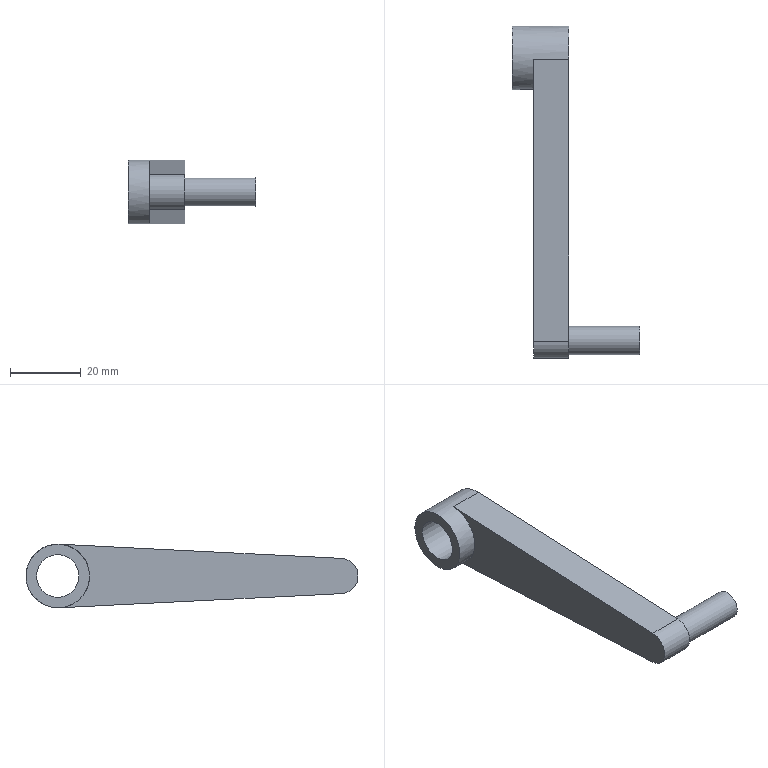Component | NX | HANDLE | 1 solid | 10 faces | box 36 x 94 x 18 mm | volume 13602 mm3 | plane 6 | cylinder 4 | commonest cylinder face diameters 18 x1 12 x1 10 x1 8 x1
STEP:
#1=CARTESIAN_POINT('',(0.,0.,0.));
#2=DIRECTION('',(0.,0.,1.));
#3=DIRECTION('',(1.,0.,0.));
#4=AXIS2_PLACEMENT_3D('',#1,#2,#3);
#5=CARTESIAN_POINT('',(764.009,-150.752,-1316.489));
#6=VERTEX_POINT('',#5);
#7=CARTESIAN_POINT('',(764.009,-159.302,-1307.5));
#8=VERTEX_POINT('',#7);
#9=CARTESIAN_POINT('',(764.009,-150.302,-1307.5));
#10=DIRECTION('',(-1.,0.,0.));
#11=DIRECTION('',(0.,-1.,0.));
#12=AXIS2_PLACEMENT_3D('',#9,#10,#11);
#13=CIRCLE('',#12,9.);
#14=CARTESIAN_POINT('',(764.009,-150.302,-1307.5));
#15=DIRECTION('',(1.,0.,0.));
#16=DIRECTION('',(0.,1.,0.));
#17=AXIS2_PLACEMENT_3D('',#14,#15,#16);
#18=CYLINDRICAL_SURFACE('',#17,9.);
#19=CARTESIAN_POINT('',(15.708,0.));
#20=DIRECTION('',(-1.,0.));
#21=VECTOR('',#20,1.);
#22=LINE('',#19,#21);
#23=(GEOMETRIC_REPRESENTATION_CONTEXT(2)PARAMETRIC_REPRESENTATION_CONTEXT()REPRESENTATION_CONTEXT('',''));
#24=DEFINITIONAL_REPRESENTATION('',(#22),#23);
#25=PCURVE('',#18,#24);
#26=CARTESIAN_POINT('',(764.009,-150.302,-1307.5));
#27=DIRECTION('',(-1.,0.,0.));
#28=DIRECTION('',(0.,-1.,0.));
#29=AXIS2_PLACEMENT_3D('',#26,#27,#28);
#30=PLANE('',#29);
#31=CARTESIAN_POINT('',(0.,0.));
#32=DIRECTION('',(1.,0.));
#33=AXIS2_PLACEMENT_2D('',#31,#32);
#34=CIRCLE('',#33,9.);
#35=(GEOMETRIC_REPRESENTATION_CONTEXT(2)PARAMETRIC_REPRESENTATION_CONTEXT()REPRESENTATION_CONTEXT('',''));
#36=DEFINITIONAL_REPRESENTATION('',(#34),#35);
#37=PCURVE('',#30,#36);
#38=SURFACE_CURVE('',#13,(#25,#37),.PCURVE_S1.);
#39=EDGE_CURVE('',#6,#8,#38,.T.);
#40=ORIENTED_EDGE('',*,*,#39,.F.);
#41=CARTESIAN_POINT('',(770.009,-150.752,-1316.489));
#42=VERTEX_POINT('',#41);
#43=CARTESIAN_POINT('',(764.009,-150.752,-1316.489));
#44=CARTESIAN_POINT('',(770.009,-150.752,-1316.489));
#45=B_SPLINE_CURVE_WITH_KNOTS('',1,(#43,#44),.UNSPECIFIED.,.F.,.F.,(2,2),(0.,6.),.PIECEWISE_BEZIER_KNOTS.);
#46=CARTESIAN_POINT('',(10.946,0.));
#47=DIRECTION('',(0.,1.));
#48=VECTOR('',#47,1.);
#49=LINE('',#46,#48);
#50=(GEOMETRIC_REPRESENTATION_CONTEXT(2)PARAMETRIC_REPRESENTATION_CONTEXT()REPRESENTATION_CONTEXT('',''));
#51=DEFINITIONAL_REPRESENTATION('',(#49),#50);
#52=PCURVE('',#18,#51);
#53=CARTESIAN_POINT('',(4.662,0.));
#54=DIRECTION('',(0.,1.));
#55=VECTOR('',#54,1.);
#56=LINE('',#53,#55);
#57=(GEOMETRIC_REPRESENTATION_CONTEXT(2)PARAMETRIC_REPRESENTATION_CONTEXT()REPRESENTATION_CONTEXT('',''));
#58=DEFINITIONAL_REPRESENTATION('',(#56),#57);
#59=PCURVE('',#18,#58);
#60=SEAM_CURVE('',#45,(#52,#59),.PCURVE_S1.);
#61=EDGE_CURVE('',#6,#42,#60,.T.);
#62=ORIENTED_EDGE('',*,*,#61,.T.);
#63=CARTESIAN_POINT('',(770.009,-150.752,-1298.511));
#64=VERTEX_POINT('',#63);
#65=CARTESIAN_POINT('',(770.009,-150.302,-1307.5));
#66=DIRECTION('',(1.,0.,0.));
#67=DIRECTION('',(0.,-1.,0.));
#68=AXIS2_PLACEMENT_3D('',#65,#66,#67);
#69=CIRCLE('',#68,9.);
#70=CARTESIAN_POINT('',(3.142,6.));
#71=DIRECTION('',(1.,0.));
#72=VECTOR('',#71,1.);
#73=LINE('',#70,#72);
#74=(GEOMETRIC_REPRESENTATION_CONTEXT(2)PARAMETRIC_REPRESENTATION_CONTEXT()REPRESENTATION_CONTEXT('',''));
#75=DEFINITIONAL_REPRESENTATION('',(#73),#74);
#76=PCURVE('',#18,#75);
#77=CARTESIAN_POINT('',(770.009,-150.302,-1307.5));
#78=DIRECTION('',(1.,0.,0.));
#79=DIRECTION('',(0.,1.,0.));
#80=AXIS2_PLACEMENT_3D('',#77,#78,#79);
#81=PLANE('',#80);
#82=CARTESIAN_POINT('',(0.,0.));
#83=DIRECTION('',(-1.,0.));
#84=AXIS2_PLACEMENT_2D('',#82,#83);
#85=CIRCLE('',#84,9.);
#86=(GEOMETRIC_REPRESENTATION_CONTEXT(2)PARAMETRIC_REPRESENTATION_CONTEXT()REPRESENTATION_CONTEXT('',''));
#87=DEFINITIONAL_REPRESENTATION('',(#85),#86);
#88=PCURVE('',#81,#87);
#89=SURFACE_CURVE('',#69,(#76,#88),.PCURVE_S1.);
#90=EDGE_CURVE('',#64,#42,#89,.T.);
#91=ORIENTED_EDGE('',*,*,#90,.F.);
#92=CARTESIAN_POINT('',(780.009,-150.752,-1298.511));
#93=VERTEX_POINT('',#92);
#94=CARTESIAN_POINT('',(770.009,-150.752,-1298.511));
#95=DIRECTION('',(1.,0.,0.));
#96=VECTOR('',#95,1.);
#97=LINE('',#94,#96);
#98=CARTESIAN_POINT('',(7.904,6.));
#99=DIRECTION('',(0.,1.));
#100=VECTOR('',#99,1.);
#101=LINE('',#98,#100);
#102=(GEOMETRIC_REPRESENTATION_CONTEXT(2)PARAMETRIC_REPRESENTATION_CONTEXT()REPRESENTATION_CONTEXT('',''));
#103=DEFINITIONAL_REPRESENTATION('',(#101),#102);
#104=PCURVE('',#18,#103);
#105=CARTESIAN_POINT('',(770.009,-230.552,-1302.506));
#106=DIRECTION('',(0.,0.05,-0.9987));
#107=DIRECTION('',(0.,-0.9987,-0.05));
#108=AXIS2_PLACEMENT_3D('',#105,#106,#107);
#109=PLANE('',#108);
#110=CARTESIAN_POINT('',(-79.9,0.));
#111=DIRECTION('',(0.,-1.));
#112=VECTOR('',#111,1.);
#113=LINE('',#110,#112);
#114=(GEOMETRIC_REPRESENTATION_CONTEXT(2)PARAMETRIC_REPRESENTATION_CONTEXT()REPRESENTATION_CONTEXT('',''));
#115=DEFINITIONAL_REPRESENTATION('',(#113),#114);
#116=PCURVE('',#109,#115);
#117=SURFACE_CURVE('',#97,(#104,#116),.PCURVE_S1.);
#118=EDGE_CURVE('',#64,#93,#117,.T.);
#119=ORIENTED_EDGE('',*,*,#118,.T.);
#120=CARTESIAN_POINT('',(780.009,-150.752,-1316.489));
#121=VERTEX_POINT('',#120);
#122=CARTESIAN_POINT('',(780.009,-150.302,-1307.5));
#123=DIRECTION('',(-1.,0.,0.));
#124=DIRECTION('',(0.,-1.,0.));
#125=AXIS2_PLACEMENT_3D('',#122,#123,#124);
#126=CIRCLE('',#125,9.);
#127=CARTESIAN_POINT('',(9.425,16.));
#128=DIRECTION('',(-1.,0.));
#129=VECTOR('',#128,1.);
#130=LINE('',#127,#129);
#131=(GEOMETRIC_REPRESENTATION_CONTEXT(2)PARAMETRIC_REPRESENTATION_CONTEXT()REPRESENTATION_CONTEXT('',''));
#132=DEFINITIONAL_REPRESENTATION('',(#130),#131);
#133=PCURVE('',#18,#132);
#134=CARTESIAN_POINT('',(780.009,-150.302,-1307.5));
#135=DIRECTION('',(-1.,0.,0.));
#136=DIRECTION('',(0.,-1.,0.));
#137=AXIS2_PLACEMENT_3D('',#134,#135,#136);
#138=PLANE('',#137);
#139=CARTESIAN_POINT('',(0.,0.));
#140=DIRECTION('',(1.,0.));
#141=AXIS2_PLACEMENT_2D('',#139,#140);
#142=CIRCLE('',#141,9.);
#143=(GEOMETRIC_REPRESENTATION_CONTEXT(2)PARAMETRIC_REPRESENTATION_CONTEXT()REPRESENTATION_CONTEXT('',''));
#144=DEFINITIONAL_REPRESENTATION('',(#142),#143);
#145=PCURVE('',#138,#144);
#146=SURFACE_CURVE('',#126,(#133,#145),.PCURVE_S1.);
#147=EDGE_CURVE('',#93,#121,#146,.T.);
#148=ORIENTED_EDGE('',*,*,#147,.T.);
#149=CARTESIAN_POINT('',(770.009,-150.752,-1316.489));
#150=DIRECTION('',(1.,0.,0.));
#151=VECTOR('',#150,1.);
#152=LINE('',#149,#151);
#153=CARTESIAN_POINT('',(4.662,6.));
#154=DIRECTION('',(0.,1.));
#155=VECTOR('',#154,1.);
#156=LINE('',#153,#155);
#157=(GEOMETRIC_REPRESENTATION_CONTEXT(2)PARAMETRIC_REPRESENTATION_CONTEXT()REPRESENTATION_CONTEXT('',''));
#158=DEFINITIONAL_REPRESENTATION('',(#156),#157);
#159=PCURVE('',#18,#158);
#160=CARTESIAN_POINT('',(770.009,-150.752,-1316.489));
#161=DIRECTION('',(0.,0.05,0.9987));
#162=DIRECTION('',(0.,0.9987,-0.05));
#163=AXIS2_PLACEMENT_3D('',#160,#161,#162);
#164=PLANE('',#163);
#165=CARTESIAN_POINT('',(-0.,0.));
#166=DIRECTION('',(0.,-1.));
#167=VECTOR('',#166,1.);
#168=LINE('',#165,#167);
#169=(GEOMETRIC_REPRESENTATION_CONTEXT(2)PARAMETRIC_REPRESENTATION_CONTEXT()REPRESENTATION_CONTEXT('',''));
#170=DEFINITIONAL_REPRESENTATION('',(#168),#169);
#171=PCURVE('',#164,#170);
#172=SURFACE_CURVE('',#152,(#159,#171),.PCURVE_S1.);
#173=EDGE_CURVE('',#42,#121,#172,.T.);
#174=ORIENTED_EDGE('',*,*,#173,.F.);
#175=ORIENTED_EDGE('',*,*,#61,.F.);
#176=CARTESIAN_POINT('',(764.009,-150.302,-1307.5));
#177=DIRECTION('',(-1.,0.,0.));
#178=DIRECTION('',(0.,-1.,0.));
#179=AXIS2_PLACEMENT_3D('',#176,#177,#178);
#180=CIRCLE('',#179,9.);
#181=CARTESIAN_POINT('',(9.425,0.));
#182=DIRECTION('',(-1.,0.));
#183=VECTOR('',#182,1.);
#184=LINE('',#181,#183);
#185=(GEOMETRIC_REPRESENTATION_CONTEXT(2)PARAMETRIC_REPRESENTATION_CONTEXT()REPRESENTATION_CONTEXT('',''));
#186=DEFINITIONAL_REPRESENTATION('',(#184),#185);
#187=PCURVE('',#18,#186);
#188=CARTESIAN_POINT('',(0.,0.));
#189=DIRECTION('',(1.,0.));
#190=AXIS2_PLACEMENT_2D('',#188,#189);
#191=CIRCLE('',#190,9.);
#192=(GEOMETRIC_REPRESENTATION_CONTEXT(2)PARAMETRIC_REPRESENTATION_CONTEXT()REPRESENTATION_CONTEXT('',''));
#193=DEFINITIONAL_REPRESENTATION('',(#191),#192);
#194=PCURVE('',#30,#193);
#195=SURFACE_CURVE('',#180,(#187,#194),.PCURVE_S1.);
#196=EDGE_CURVE('',#8,#6,#195,.T.);
#197=ORIENTED_EDGE('',*,*,#196,.F.);
#198=EDGE_LOOP('',(#40,#62,#91,#119,#148,#174,#175,#197));
#199=FACE_BOUND('',#198,.T.);
#200=ADVANCED_FACE('',(#199),#18,.T.);
#201=CARTESIAN_POINT('',(764.009,-156.302,-1307.5));
#202=VERTEX_POINT('',#201);
#203=CARTESIAN_POINT('',(764.009,-150.302,-1307.5));
#204=DIRECTION('',(-1.,0.,0.));
#205=DIRECTION('',(0.,-1.,0.));
#206=AXIS2_PLACEMENT_3D('',#203,#204,#205);
#207=CIRCLE('',#206,6.);
#208=CARTESIAN_POINT('',(764.009,-150.302,-1307.5));
#209=DIRECTION('',(1.,0.,0.));
#210=DIRECTION('',(0.,1.,0.));
#211=AXIS2_PLACEMENT_3D('',#208,#209,#210);
#212=CYLINDRICAL_SURFACE('',#211,6.);
#213=CARTESIAN_POINT('',(9.425,0.));
#214=DIRECTION('',(-1.,0.));
#215=VECTOR('',#214,1.);
#216=LINE('',#213,#215);
#217=(GEOMETRIC_REPRESENTATION_CONTEXT(2)PARAMETRIC_REPRESENTATION_CONTEXT()REPRESENTATION_CONTEXT('',''));
#218=DEFINITIONAL_REPRESENTATION('',(#216),#217);
#219=PCURVE('',#212,#218);
#220=CARTESIAN_POINT('',(0.,0.));
#221=DIRECTION('',(1.,0.));
#222=AXIS2_PLACEMENT_2D('',#220,#221);
#223=CIRCLE('',#222,6.);
#224=(GEOMETRIC_REPRESENTATION_CONTEXT(2)PARAMETRIC_REPRESENTATION_CONTEXT()REPRESENTATION_CONTEXT('',''));
#225=DEFINITIONAL_REPRESENTATION('',(#223),#224);
#226=PCURVE('',#30,#225);
#227=SURFACE_CURVE('',#207,(#219,#226),.PCURVE_S1.);
#228=EDGE_CURVE('',#202,#202,#227,.T.);
#229=ORIENTED_EDGE('',*,*,#228,.F.);
#230=CARTESIAN_POINT('',(780.009,-156.302,-1307.5));
#231=VERTEX_POINT('',#230);
#232=CARTESIAN_POINT('',(764.009,-156.302,-1307.5));
#233=CARTESIAN_POINT('',(780.009,-156.302,-1307.5));
#234=B_SPLINE_CURVE_WITH_KNOTS('',1,(#232,#233),.UNSPECIFIED.,.F.,.F.,(2,2),(0.,16.),.PIECEWISE_BEZIER_KNOTS.);
#235=CARTESIAN_POINT('',(9.425,0.));
#236=DIRECTION('',(0.,1.));
#237=VECTOR('',#236,1.);
#238=LINE('',#235,#237);
#239=(GEOMETRIC_REPRESENTATION_CONTEXT(2)PARAMETRIC_REPRESENTATION_CONTEXT()REPRESENTATION_CONTEXT('',''));
#240=DEFINITIONAL_REPRESENTATION('',(#238),#239);
#241=PCURVE('',#212,#240);
#242=CARTESIAN_POINT('',(3.142,0.));
#243=DIRECTION('',(0.,1.));
#244=VECTOR('',#243,1.);
#245=LINE('',#242,#244);
#246=(GEOMETRIC_REPRESENTATION_CONTEXT(2)PARAMETRIC_REPRESENTATION_CONTEXT()REPRESENTATION_CONTEXT('',''));
#247=DEFINITIONAL_REPRESENTATION('',(#245),#246);
#248=PCURVE('',#212,#247);
#249=SEAM_CURVE('',#234,(#241,#248),.PCURVE_S1.);
#250=EDGE_CURVE('',#202,#231,#249,.T.);
#251=ORIENTED_EDGE('',*,*,#250,.T.);
#252=CARTESIAN_POINT('',(780.009,-150.302,-1307.5));
#253=DIRECTION('',(-1.,0.,0.));
#254=DIRECTION('',(0.,-1.,0.));
#255=AXIS2_PLACEMENT_3D('',#252,#253,#254);
#256=CIRCLE('',#255,6.);
#257=CARTESIAN_POINT('',(9.425,16.));
#258=DIRECTION('',(-1.,0.));
#259=VECTOR('',#258,1.);
#260=LINE('',#257,#259);
#261=(GEOMETRIC_REPRESENTATION_CONTEXT(2)PARAMETRIC_REPRESENTATION_CONTEXT()REPRESENTATION_CONTEXT('',''));
#262=DEFINITIONAL_REPRESENTATION('',(#260),#261);
#263=PCURVE('',#212,#262);
#264=CARTESIAN_POINT('',(0.,0.));
#265=DIRECTION('',(1.,0.));
#266=AXIS2_PLACEMENT_2D('',#264,#265);
#267=CIRCLE('',#266,6.);
#268=(GEOMETRIC_REPRESENTATION_CONTEXT(2)PARAMETRIC_REPRESENTATION_CONTEXT()REPRESENTATION_CONTEXT('',''));
#269=DEFINITIONAL_REPRESENTATION('',(#267),#268);
#270=PCURVE('',#138,#269);
#271=SURFACE_CURVE('',#256,(#263,#270),.PCURVE_S1.);
#272=EDGE_CURVE('',#231,#231,#271,.T.);
#273=ORIENTED_EDGE('',*,*,#272,.T.);
#274=ORIENTED_EDGE('',*,*,#250,.F.);
#275=EDGE_LOOP('',(#229,#251,#273,#274));
#276=FACE_BOUND('',#275,.F.);
#277=ADVANCED_FACE('',(#276),#212,.F.);
#278=ORIENTED_EDGE('',*,*,#196,.T.);
#279=ORIENTED_EDGE('',*,*,#39,.T.);
#280=EDGE_LOOP('',(#278,#279));
#281=FACE_BOUND('',#280,.T.);
#282=ORIENTED_EDGE('',*,*,#228,.F.);
#283=EDGE_LOOP('',(#282));
#284=FACE_BOUND('',#283,.T.);
#285=ADVANCED_FACE('',(#281,#284),#30,.T.);
#286=CARTESIAN_POINT('',(780.009,-234.302,-1307.5));
#287=VERTEX_POINT('',#286);
#288=CARTESIAN_POINT('',(780.009,-230.302,-1307.5));
#289=DIRECTION('',(1.,0.,0.));
#290=DIRECTION('',(0.,-1.,0.));
#291=AXIS2_PLACEMENT_3D('',#288,#289,#290);
#292=CIRCLE('',#291,4.);
#293=CARTESIAN_POINT('',(84.,0.));
#294=CARTESIAN_POINT('',(84.,-6.928));
#295=CARTESIAN_POINT('',(78.,-3.464));
#296=CARTESIAN_POINT('',(72.,-0.));
#297=CARTESIAN_POINT('',(78.,3.464));
#298=CARTESIAN_POINT('',(84.,6.928));
#299=CARTESIAN_POINT('',(84.,0.));
#300=(BOUNDED_CURVE()B_SPLINE_CURVE(2,(#293,#294,#295,#296,#297,#298,#299),.UNSPECIFIED.,.T.,.F.)B_SPLINE_CURVE_WITH_KNOTS((1,2,2,2,2,1),(-2.094,0.,2.094,4.189,6.283,8.378),.UNSPECIFIED.)CURVE()GEOMETRIC_REPRESENTATION_ITEM()RATIONAL_B_SPLINE_CURVE((1.,0.5,1.,0.5,1.,0.5,1.))REPRESENTATION_ITEM(''));
#301=(GEOMETRIC_REPRESENTATION_CONTEXT(2)PARAMETRIC_REPRESENTATION_CONTEXT()REPRESENTATION_CONTEXT('',''));
#302=DEFINITIONAL_REPRESENTATION('',(#300),#301);
#303=PCURVE('',#138,#302);
#304=CARTESIAN_POINT('',(800.009,-230.302,-1307.5));
#305=DIRECTION('',(-1.,0.,0.));
#306=DIRECTION('',(0.,-1.,0.));
#307=AXIS2_PLACEMENT_3D('',#304,#305,#306);
#308=CYLINDRICAL_SURFACE('',#307,4.);
#309=CARTESIAN_POINT('',(6.283,20.));
#310=DIRECTION('',(-1.,0.));
#311=VECTOR('',#310,1.);
#312=LINE('',#309,#311);
#313=(GEOMETRIC_REPRESENTATION_CONTEXT(2)PARAMETRIC_REPRESENTATION_CONTEXT()REPRESENTATION_CONTEXT('',''));
#314=DEFINITIONAL_REPRESENTATION('',(#312),#313);
#315=PCURVE('',#308,#314);
#316=SURFACE_CURVE('',#292,(#303,#315),.PCURVE_S1.);
#317=EDGE_CURVE('',#287,#287,#316,.T.);
#318=ORIENTED_EDGE('',*,*,#317,.F.);
#319=EDGE_LOOP('',(#318));
#320=FACE_BOUND('',#319,.T.);
#321=ORIENTED_EDGE('',*,*,#147,.F.);
#322=CARTESIAN_POINT('',(780.009,-230.552,-1302.506));
#323=VERTEX_POINT('',#322);
#324=CARTESIAN_POINT('',(780.009,-230.552,-1302.506));
#325=DIRECTION('',(0.,0.9987,0.05));
#326=VECTOR('',#325,1.);
#327=LINE('',#324,#326);
#328=CARTESIAN_POINT('',(80.25,4.994));
#329=DIRECTION('',(-0.9987,0.05));
#330=VECTOR('',#329,1.);
#331=LINE('',#328,#330);
#332=(GEOMETRIC_REPRESENTATION_CONTEXT(2)PARAMETRIC_REPRESENTATION_CONTEXT()REPRESENTATION_CONTEXT('',''));
#333=DEFINITIONAL_REPRESENTATION('',(#331),#332);
#334=PCURVE('',#138,#333);
#335=CARTESIAN_POINT('',(0.,-10.));
#336=DIRECTION('',(-1.,0.));
#337=VECTOR('',#336,1.);
#338=LINE('',#335,#337);
#339=(GEOMETRIC_REPRESENTATION_CONTEXT(2)PARAMETRIC_REPRESENTATION_CONTEXT()REPRESENTATION_CONTEXT('',''));
#340=DEFINITIONAL_REPRESENTATION('',(#338),#339);
#341=PCURVE('',#109,#340);
#342=SURFACE_CURVE('',#327,(#334,#341),.PCURVE_S1.);
#343=EDGE_CURVE('',#323,#93,#342,.T.);
#344=ORIENTED_EDGE('',*,*,#343,.F.);
#345=CARTESIAN_POINT('',(780.009,-230.552,-1312.494));
#346=VERTEX_POINT('',#345);
#347=CARTESIAN_POINT('',(780.009,-230.302,-1307.5));
#348=DIRECTION('',(-1.,0.,0.));
#349=DIRECTION('',(0.,-1.,0.));
#350=AXIS2_PLACEMENT_3D('',#347,#348,#349);
#351=CIRCLE('',#350,5.);
#352=CARTESIAN_POINT('',(80.,0.));
#353=DIRECTION('',(1.,0.));
#354=AXIS2_PLACEMENT_2D('',#352,#353);
#355=CIRCLE('',#354,5.);
#356=(GEOMETRIC_REPRESENTATION_CONTEXT(2)PARAMETRIC_REPRESENTATION_CONTEXT()REPRESENTATION_CONTEXT('',''));
#357=DEFINITIONAL_REPRESENTATION('',(#355),#356);
#358=PCURVE('',#138,#357);
#359=CARTESIAN_POINT('',(770.009,-230.302,-1307.5));
#360=DIRECTION('',(1.,0.,0.));
#361=DIRECTION('',(0.,1.,0.));
#362=AXIS2_PLACEMENT_3D('',#359,#360,#361);
#363=CYLINDRICAL_SURFACE('',#362,5.);
#364=CARTESIAN_POINT('',(9.425,10.));
#365=DIRECTION('',(-1.,0.));
#366=VECTOR('',#365,1.);
#367=LINE('',#364,#366);
#368=(GEOMETRIC_REPRESENTATION_CONTEXT(2)PARAMETRIC_REPRESENTATION_CONTEXT()REPRESENTATION_CONTEXT('',''));
#369=DEFINITIONAL_REPRESENTATION('',(#367),#368);
#370=PCURVE('',#363,#369);
#371=SURFACE_CURVE('',#351,(#358,#370),.PCURVE_S1.);
#372=EDGE_CURVE('',#346,#323,#371,.T.);
#373=ORIENTED_EDGE('',*,*,#372,.F.);
#374=CARTESIAN_POINT('',(780.009,-150.752,-1316.489));
#375=DIRECTION('',(0.,-0.9987,0.05));
#376=VECTOR('',#375,1.);
#377=LINE('',#374,#376);
#378=CARTESIAN_POINT('',(0.45,-8.989));
#379=DIRECTION('',(0.9987,0.05));
#380=VECTOR('',#379,1.);
#381=LINE('',#378,#380);
#382=(GEOMETRIC_REPRESENTATION_CONTEXT(2)PARAMETRIC_REPRESENTATION_CONTEXT()REPRESENTATION_CONTEXT('',''));
#383=DEFINITIONAL_REPRESENTATION('',(#381),#382);
#384=PCURVE('',#138,#383);
#385=CARTESIAN_POINT('',(0.,-10.));
#386=DIRECTION('',(-1.,0.));
#387=VECTOR('',#386,1.);
#388=LINE('',#385,#387);
#389=(GEOMETRIC_REPRESENTATION_CONTEXT(2)PARAMETRIC_REPRESENTATION_CONTEXT()REPRESENTATION_CONTEXT('',''));
#390=DEFINITIONAL_REPRESENTATION('',(#388),#389);
#391=PCURVE('',#164,#390);
#392=SURFACE_CURVE('',#377,(#384,#391),.PCURVE_S1.);
#393=EDGE_CURVE('',#121,#346,#392,.T.);
#394=ORIENTED_EDGE('',*,*,#393,.F.);
#395=EDGE_LOOP('',(#321,#344,#373,#394));
#396=FACE_BOUND('',#395,.T.);
#397=ORIENTED_EDGE('',*,*,#272,.T.);
#398=EDGE_LOOP('',(#397));
#399=FACE_BOUND('',#398,.T.);
#400=ADVANCED_FACE('',(#320,#396,#399),#138,.F.);
#401=ORIENTED_EDGE('',*,*,#393,.T.);
#402=CARTESIAN_POINT('',(770.009,-230.552,-1312.494));
#403=VERTEX_POINT('',#402);
#404=CARTESIAN_POINT('',(770.009,-230.552,-1312.494));
#405=DIRECTION('',(1.,0.,0.));
#406=VECTOR('',#405,1.);
#407=LINE('',#404,#406);
#408=CARTESIAN_POINT('',(-79.9,0.));
#409=DIRECTION('',(0.,-1.));
#410=VECTOR('',#409,1.);
#411=LINE('',#408,#410);
#412=(GEOMETRIC_REPRESENTATION_CONTEXT(2)PARAMETRIC_REPRESENTATION_CONTEXT()REPRESENTATION_CONTEXT('',''));
#413=DEFINITIONAL_REPRESENTATION('',(#411),#412);
#414=PCURVE('',#164,#413);
#415=CARTESIAN_POINT('',(4.662,0.));
#416=DIRECTION('',(0.,1.));
#417=VECTOR('',#416,1.);
#418=LINE('',#415,#417);
#419=(GEOMETRIC_REPRESENTATION_CONTEXT(2)PARAMETRIC_REPRESENTATION_CONTEXT()REPRESENTATION_CONTEXT('',''));
#420=DEFINITIONAL_REPRESENTATION('',(#418),#419);
#421=PCURVE('',#363,#420);
#422=SURFACE_CURVE('',#407,(#414,#421),.PCURVE_S1.);
#423=EDGE_CURVE('',#403,#346,#422,.T.);
#424=ORIENTED_EDGE('',*,*,#423,.F.);
#425=CARTESIAN_POINT('',(770.009,-150.752,-1316.489));
#426=DIRECTION('',(0.,-0.9987,0.05));
#427=VECTOR('',#426,1.);
#428=LINE('',#425,#427);
#429=CARTESIAN_POINT('',(0.,0.));
#430=DIRECTION('',(-1.,0.));
#431=VECTOR('',#430,1.);
#432=LINE('',#429,#431);
#433=(GEOMETRIC_REPRESENTATION_CONTEXT(2)PARAMETRIC_REPRESENTATION_CONTEXT()REPRESENTATION_CONTEXT('',''));
#434=DEFINITIONAL_REPRESENTATION('',(#432),#433);
#435=PCURVE('',#164,#434);
#436=CARTESIAN_POINT('',(-0.45,-8.989));
#437=DIRECTION('',(-0.9987,0.05));
#438=VECTOR('',#437,1.);
#439=LINE('',#436,#438);
#440=(GEOMETRIC_REPRESENTATION_CONTEXT(2)PARAMETRIC_REPRESENTATION_CONTEXT()REPRESENTATION_CONTEXT('',''));
#441=DEFINITIONAL_REPRESENTATION('',(#439),#440);
#442=PCURVE('',#81,#441);
#443=SURFACE_CURVE('',#428,(#435,#442),.PCURVE_S1.);
#444=EDGE_CURVE('',#42,#403,#443,.T.);
#445=ORIENTED_EDGE('',*,*,#444,.F.);
#446=ORIENTED_EDGE('',*,*,#173,.T.);
#447=EDGE_LOOP('',(#401,#424,#445,#446));
#448=FACE_BOUND('',#447,.T.);
#449=ADVANCED_FACE('',(#448),#164,.F.);
#450=ORIENTED_EDGE('',*,*,#372,.T.);
#451=CARTESIAN_POINT('',(770.009,-230.552,-1302.506));
#452=VERTEX_POINT('',#451);
#453=CARTESIAN_POINT('',(770.009,-230.552,-1302.506));
#454=DIRECTION('',(1.,0.,0.));
#455=VECTOR('',#454,1.);
#456=LINE('',#453,#455);
#457=CARTESIAN_POINT('',(1.621,0.));
#458=DIRECTION('',(0.,1.));
#459=VECTOR('',#458,1.);
#460=LINE('',#457,#459);
#461=(GEOMETRIC_REPRESENTATION_CONTEXT(2)PARAMETRIC_REPRESENTATION_CONTEXT()REPRESENTATION_CONTEXT('',''));
#462=DEFINITIONAL_REPRESENTATION('',(#460),#461);
#463=PCURVE('',#363,#462);
#464=CARTESIAN_POINT('',(0.,0.));
#465=DIRECTION('',(0.,-1.));
#466=VECTOR('',#465,1.);
#467=LINE('',#464,#466);
#468=(GEOMETRIC_REPRESENTATION_CONTEXT(2)PARAMETRIC_REPRESENTATION_CONTEXT()REPRESENTATION_CONTEXT('',''));
#469=DEFINITIONAL_REPRESENTATION('',(#467),#468);
#470=PCURVE('',#109,#469);
#471=SURFACE_CURVE('',#456,(#463,#470),.PCURVE_S1.);
#472=EDGE_CURVE('',#452,#323,#471,.T.);
#473=ORIENTED_EDGE('',*,*,#472,.F.);
#474=CARTESIAN_POINT('',(770.009,-230.302,-1307.5));
#475=DIRECTION('',(-1.,0.,0.));
#476=DIRECTION('',(0.,-1.,0.));
#477=AXIS2_PLACEMENT_3D('',#474,#475,#476);
#478=CIRCLE('',#477,5.);
#479=CARTESIAN_POINT('',(9.425,0.));
#480=DIRECTION('',(-1.,0.));
#481=VECTOR('',#480,1.);
#482=LINE('',#479,#481);
#483=(GEOMETRIC_REPRESENTATION_CONTEXT(2)PARAMETRIC_REPRESENTATION_CONTEXT()REPRESENTATION_CONTEXT('',''));
#484=DEFINITIONAL_REPRESENTATION('',(#482),#483);
#485=PCURVE('',#363,#484);
#486=CARTESIAN_POINT('',(-85.,0.));
#487=CARTESIAN_POINT('',(-85.,8.66));
#488=CARTESIAN_POINT('',(-77.5,4.33));
#489=CARTESIAN_POINT('',(-70.,0.));
#490=CARTESIAN_POINT('',(-77.5,-4.33));
#491=CARTESIAN_POINT('',(-85.,-8.66));
#492=CARTESIAN_POINT('',(-85.,0.));
#493=(BOUNDED_CURVE()B_SPLINE_CURVE(2,(#486,#487,#488,#489,#490,#491,#492),.UNSPECIFIED.,.T.,.F.)B_SPLINE_CURVE_WITH_KNOTS((1,2,2,2,2,1),(-2.094,0.,2.094,4.189,6.283,8.378),.UNSPECIFIED.)CURVE()GEOMETRIC_REPRESENTATION_ITEM()RATIONAL_B_SPLINE_CURVE((1.,0.5,1.,0.5,1.,0.5,1.))REPRESENTATION_ITEM(''));
#494=(GEOMETRIC_REPRESENTATION_CONTEXT(2)PARAMETRIC_REPRESENTATION_CONTEXT()REPRESENTATION_CONTEXT('',''));
#495=DEFINITIONAL_REPRESENTATION('',(#493),#494);
#496=PCURVE('',#81,#495);
#497=SURFACE_CURVE('',#478,(#485,#496),.PCURVE_S1.);
#498=EDGE_CURVE('',#403,#452,#497,.T.);
#499=ORIENTED_EDGE('',*,*,#498,.F.);
#500=ORIENTED_EDGE('',*,*,#423,.T.);
#501=EDGE_LOOP('',(#450,#473,#499,#500));
#502=FACE_BOUND('',#501,.T.);
#503=ADVANCED_FACE('',(#502),#363,.T.);
#504=ORIENTED_EDGE('',*,*,#343,.T.);
#505=ORIENTED_EDGE('',*,*,#118,.F.);
#506=CARTESIAN_POINT('',(770.009,-230.552,-1302.506));
#507=DIRECTION('',(0.,0.9987,0.05));
#508=VECTOR('',#507,1.);
#509=LINE('',#506,#508);
#510=CARTESIAN_POINT('',(0.,0.));
#511=DIRECTION('',(-1.,0.));
#512=VECTOR('',#511,1.);
#513=LINE('',#510,#512);
#514=(GEOMETRIC_REPRESENTATION_CONTEXT(2)PARAMETRIC_REPRESENTATION_CONTEXT()REPRESENTATION_CONTEXT('',''));
#515=DEFINITIONAL_REPRESENTATION('',(#513),#514);
#516=PCURVE('',#109,#515);
#517=CARTESIAN_POINT('',(-80.25,4.994));
#518=DIRECTION('',(0.9987,0.05));
#519=VECTOR('',#518,1.);
#520=LINE('',#517,#519);
#521=(GEOMETRIC_REPRESENTATION_CONTEXT(2)PARAMETRIC_REPRESENTATION_CONTEXT()REPRESENTATION_CONTEXT('',''));
#522=DEFINITIONAL_REPRESENTATION('',(#520),#521);
#523=PCURVE('',#81,#522);
#524=SURFACE_CURVE('',#509,(#516,#523),.PCURVE_S1.);
#525=EDGE_CURVE('',#452,#64,#524,.T.);
#526=ORIENTED_EDGE('',*,*,#525,.F.);
#527=ORIENTED_EDGE('',*,*,#472,.T.);
#528=EDGE_LOOP('',(#504,#505,#526,#527));
#529=FACE_BOUND('',#528,.T.);
#530=ADVANCED_FACE('',(#529),#109,.F.);
#531=ORIENTED_EDGE('',*,*,#90,.T.);
#532=ORIENTED_EDGE('',*,*,#444,.T.);
#533=ORIENTED_EDGE('',*,*,#498,.T.);
#534=ORIENTED_EDGE('',*,*,#525,.T.);
#535=EDGE_LOOP('',(#531,#532,#533,#534));
#536=FACE_BOUND('',#535,.T.);
#537=ADVANCED_FACE('',(#536),#81,.F.);
#538=CARTESIAN_POINT('',(800.009,-234.302,-1307.5));
#539=VERTEX_POINT('',#538);
#540=CARTESIAN_POINT('',(800.009,-230.302,-1307.5));
#541=DIRECTION('',(1.,0.,0.));
#542=DIRECTION('',(0.,-1.,0.));
#543=AXIS2_PLACEMENT_3D('',#540,#541,#542);
#544=CIRCLE('',#543,4.);
#545=CARTESIAN_POINT('',(6.283,0.));
#546=DIRECTION('',(-1.,0.));
#547=VECTOR('',#546,1.);
#548=LINE('',#545,#547);
#549=(GEOMETRIC_REPRESENTATION_CONTEXT(2)PARAMETRIC_REPRESENTATION_CONTEXT()REPRESENTATION_CONTEXT('',''));
#550=DEFINITIONAL_REPRESENTATION('',(#548),#549);
#551=PCURVE('',#308,#550);
#552=CARTESIAN_POINT('',(800.009,-230.302,-1307.5));
#553=DIRECTION('',(1.,0.,0.));
#554=DIRECTION('',(0.,1.,0.));
#555=AXIS2_PLACEMENT_3D('',#552,#553,#554);
#556=PLANE('',#555);
#557=CARTESIAN_POINT('',(0.,0.));
#558=DIRECTION('',(-1.,0.));
#559=AXIS2_PLACEMENT_2D('',#557,#558);
#560=CIRCLE('',#559,4.);
#561=(GEOMETRIC_REPRESENTATION_CONTEXT(2)PARAMETRIC_REPRESENTATION_CONTEXT()REPRESENTATION_CONTEXT('',''));
#562=DEFINITIONAL_REPRESENTATION('',(#560),#561);
#563=PCURVE('',#556,#562);
#564=SURFACE_CURVE('',#544,(#551,#563),.PCURVE_S1.);
#565=EDGE_CURVE('',#539,#539,#564,.T.);
#566=ORIENTED_EDGE('',*,*,#565,.F.);
#567=CARTESIAN_POINT('',(800.009,-234.302,-1307.5));
#568=CARTESIAN_POINT('',(780.009,-234.302,-1307.5));
#569=B_SPLINE_CURVE_WITH_KNOTS('',1,(#567,#568),.UNSPECIFIED.,.F.,.F.,(2,2),(0.,20.),.PIECEWISE_BEZIER_KNOTS.);
#570=CARTESIAN_POINT('',(6.283,0.));
#571=DIRECTION('',(0.,1.));
#572=VECTOR('',#571,1.);
#573=LINE('',#570,#572);
#574=(GEOMETRIC_REPRESENTATION_CONTEXT(2)PARAMETRIC_REPRESENTATION_CONTEXT()REPRESENTATION_CONTEXT('',''));
#575=DEFINITIONAL_REPRESENTATION('',(#573),#574);
#576=PCURVE('',#308,#575);
#577=CARTESIAN_POINT('',(0.,0.));
#578=DIRECTION('',(0.,1.));
#579=VECTOR('',#578,1.);
#580=LINE('',#577,#579);
#581=(GEOMETRIC_REPRESENTATION_CONTEXT(2)PARAMETRIC_REPRESENTATION_CONTEXT()REPRESENTATION_CONTEXT('',''));
#582=DEFINITIONAL_REPRESENTATION('',(#580),#581);
#583=PCURVE('',#308,#582);
#584=SEAM_CURVE('',#569,(#576,#583),.PCURVE_S1.);
#585=EDGE_CURVE('',#539,#287,#584,.T.);
#586=ORIENTED_EDGE('',*,*,#585,.T.);
#587=ORIENTED_EDGE('',*,*,#317,.T.);
#588=ORIENTED_EDGE('',*,*,#585,.F.);
#589=EDGE_LOOP('',(#566,#586,#587,#588));
#590=FACE_BOUND('',#589,.T.);
#591=ADVANCED_FACE('',(#590),#308,.T.);
#592=ORIENTED_EDGE('',*,*,#565,.T.);
#593=EDGE_LOOP('',(#592));
#594=FACE_BOUND('',#593,.T.);
#595=ADVANCED_FACE('',(#594),#556,.T.);
#596=CLOSED_SHELL('',(#200,#277,#285,#400,#449,#503,#530,#537,#591,#595));
#597=MANIFOLD_SOLID_BREP('',#596);
#598=(LENGTH_UNIT()NAMED_UNIT(*)SI_UNIT(.MILLI.,.METRE.));
#599=UNCERTAINTY_MEASURE_WITH_UNIT(LENGTH_MEASURE(0.000002),#598,'','');
#600=(NAMED_UNIT(*)PLANE_ANGLE_UNIT()SI_UNIT($,.RADIAN.));
#601=(NAMED_UNIT(*)SI_UNIT($,.STERADIAN.)SOLID_ANGLE_UNIT());
#602=(GEOMETRIC_REPRESENTATION_CONTEXT(3)GLOBAL_UNCERTAINTY_ASSIGNED_CONTEXT((#599))GLOBAL_UNIT_ASSIGNED_CONTEXT((#598,#600,#601))REPRESENTATION_CONTEXT('',''));
#603=ADVANCED_BREP_SHAPE_REPRESENTATION('',(#4,#597),#602);